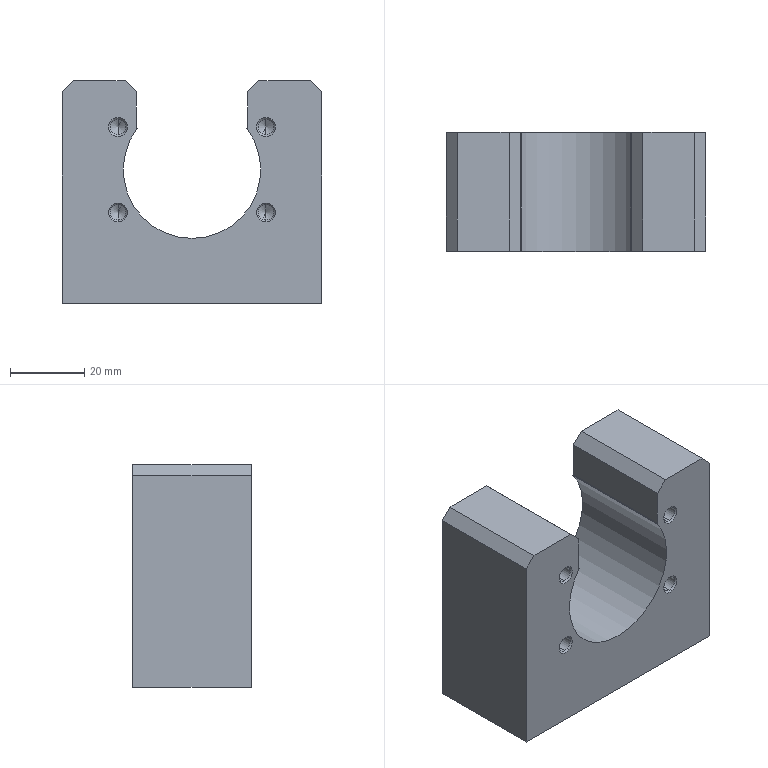CAM job | Mastercam | mm | 9 operations | part box 70 x 32 x 60
1. Facing | 20 - 63 平铣刀
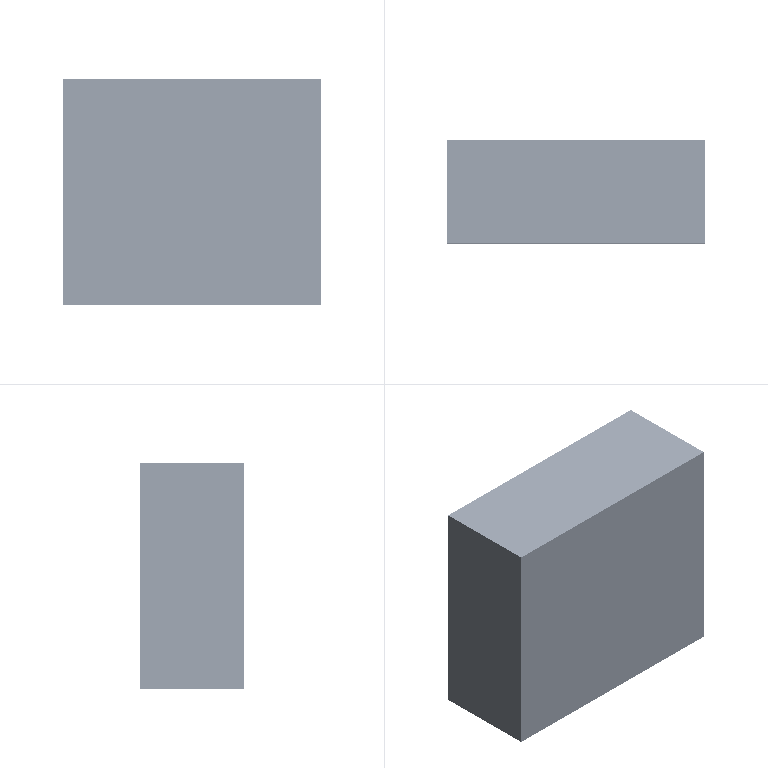2. 2D High Speed (2D Dynamic Mill) | 9 - 10 平铣刀
3. Contour (2D) | 10 - 10 平铣刀
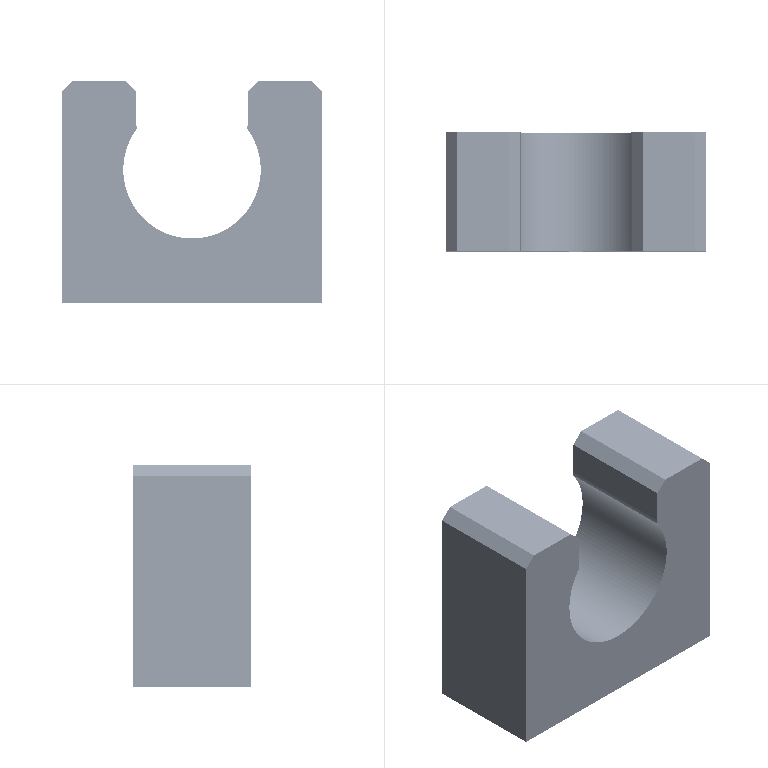4. Contour (2D chamfer) | 7 - 4 倒角刀
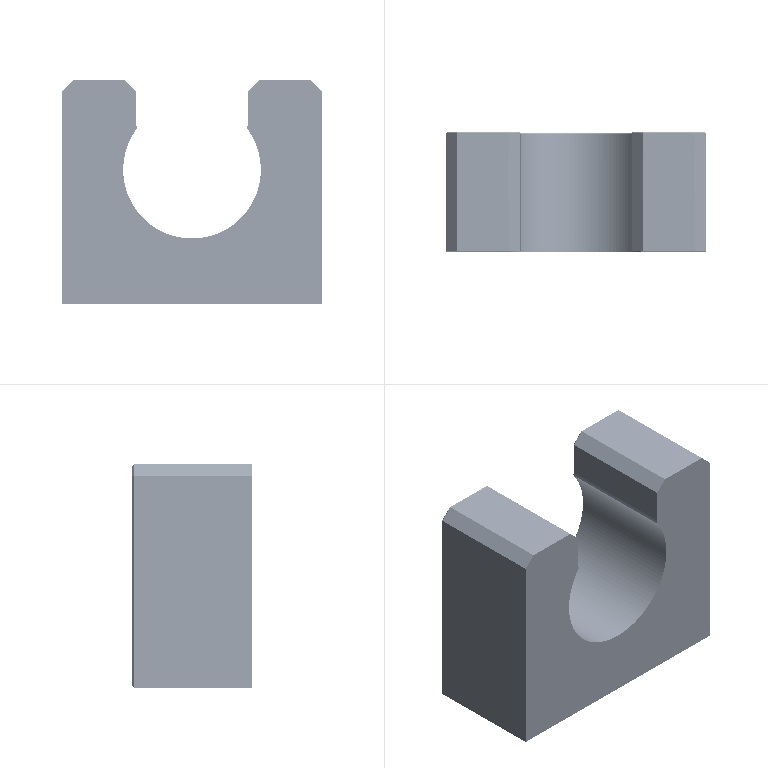5. Contour (Ramp) | 10 - 10 平铣刀
6. Facing | 20 - 63 平铣刀
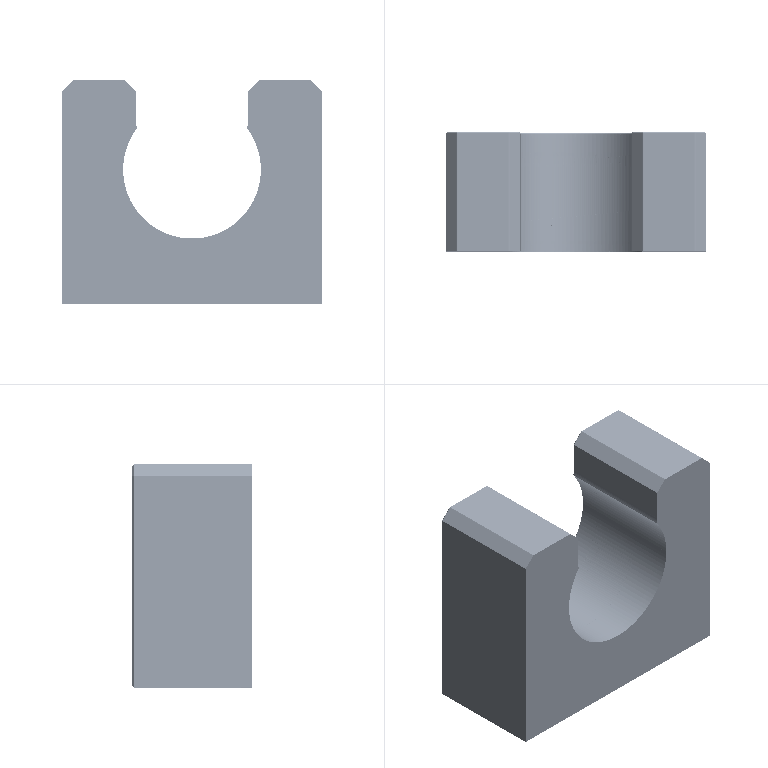7. Contour (2D chamfer) | 7 - 4 倒角刀
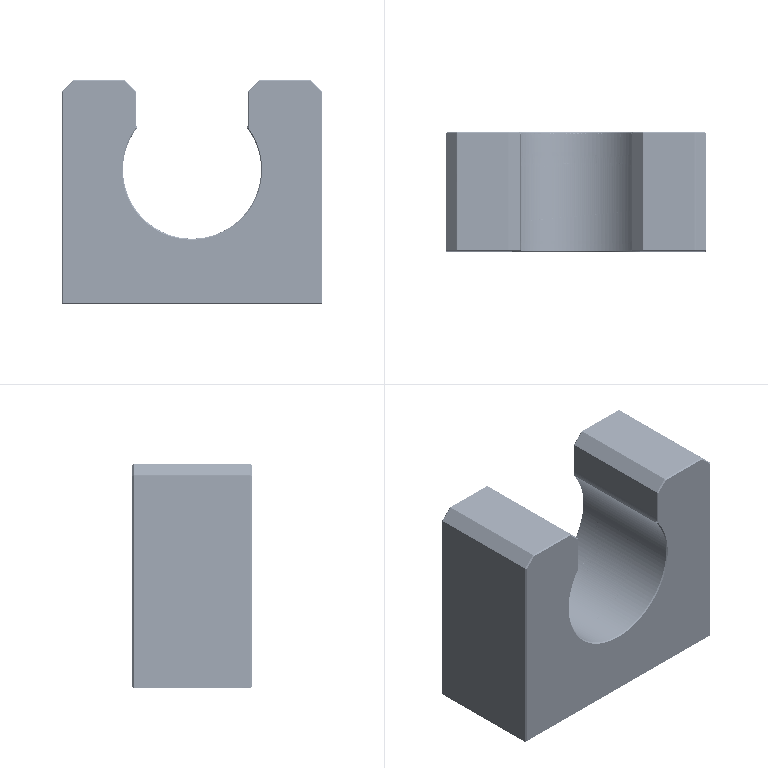8. Drill/Counterbore | 7 - 4 倒角刀
9. Drill/Counterbore | 7 - 4 倒角刀